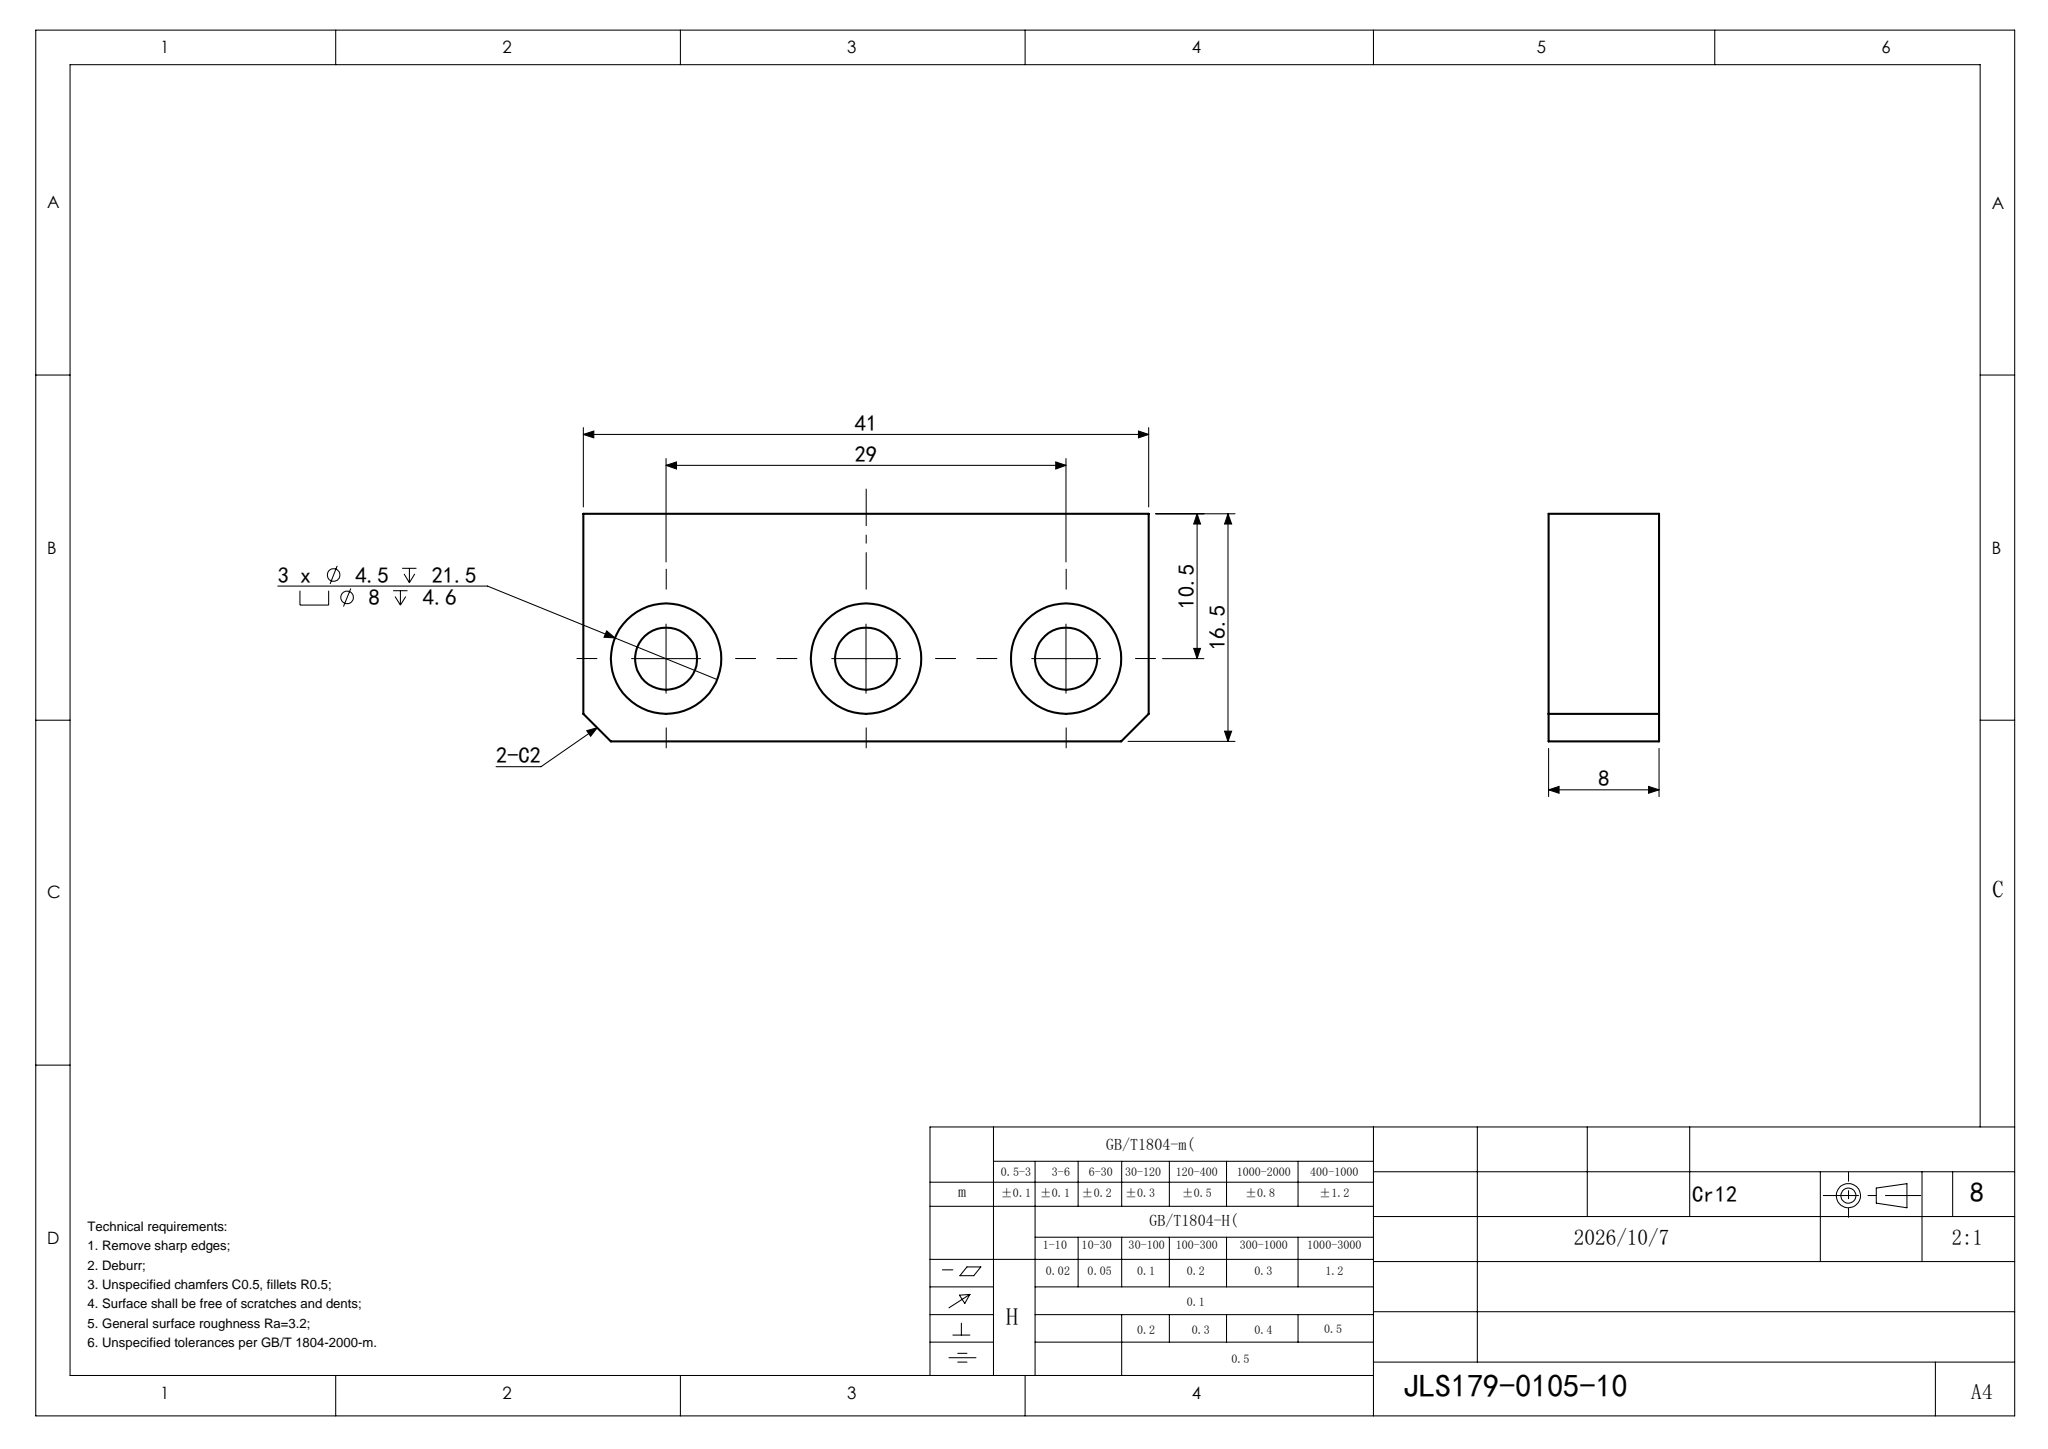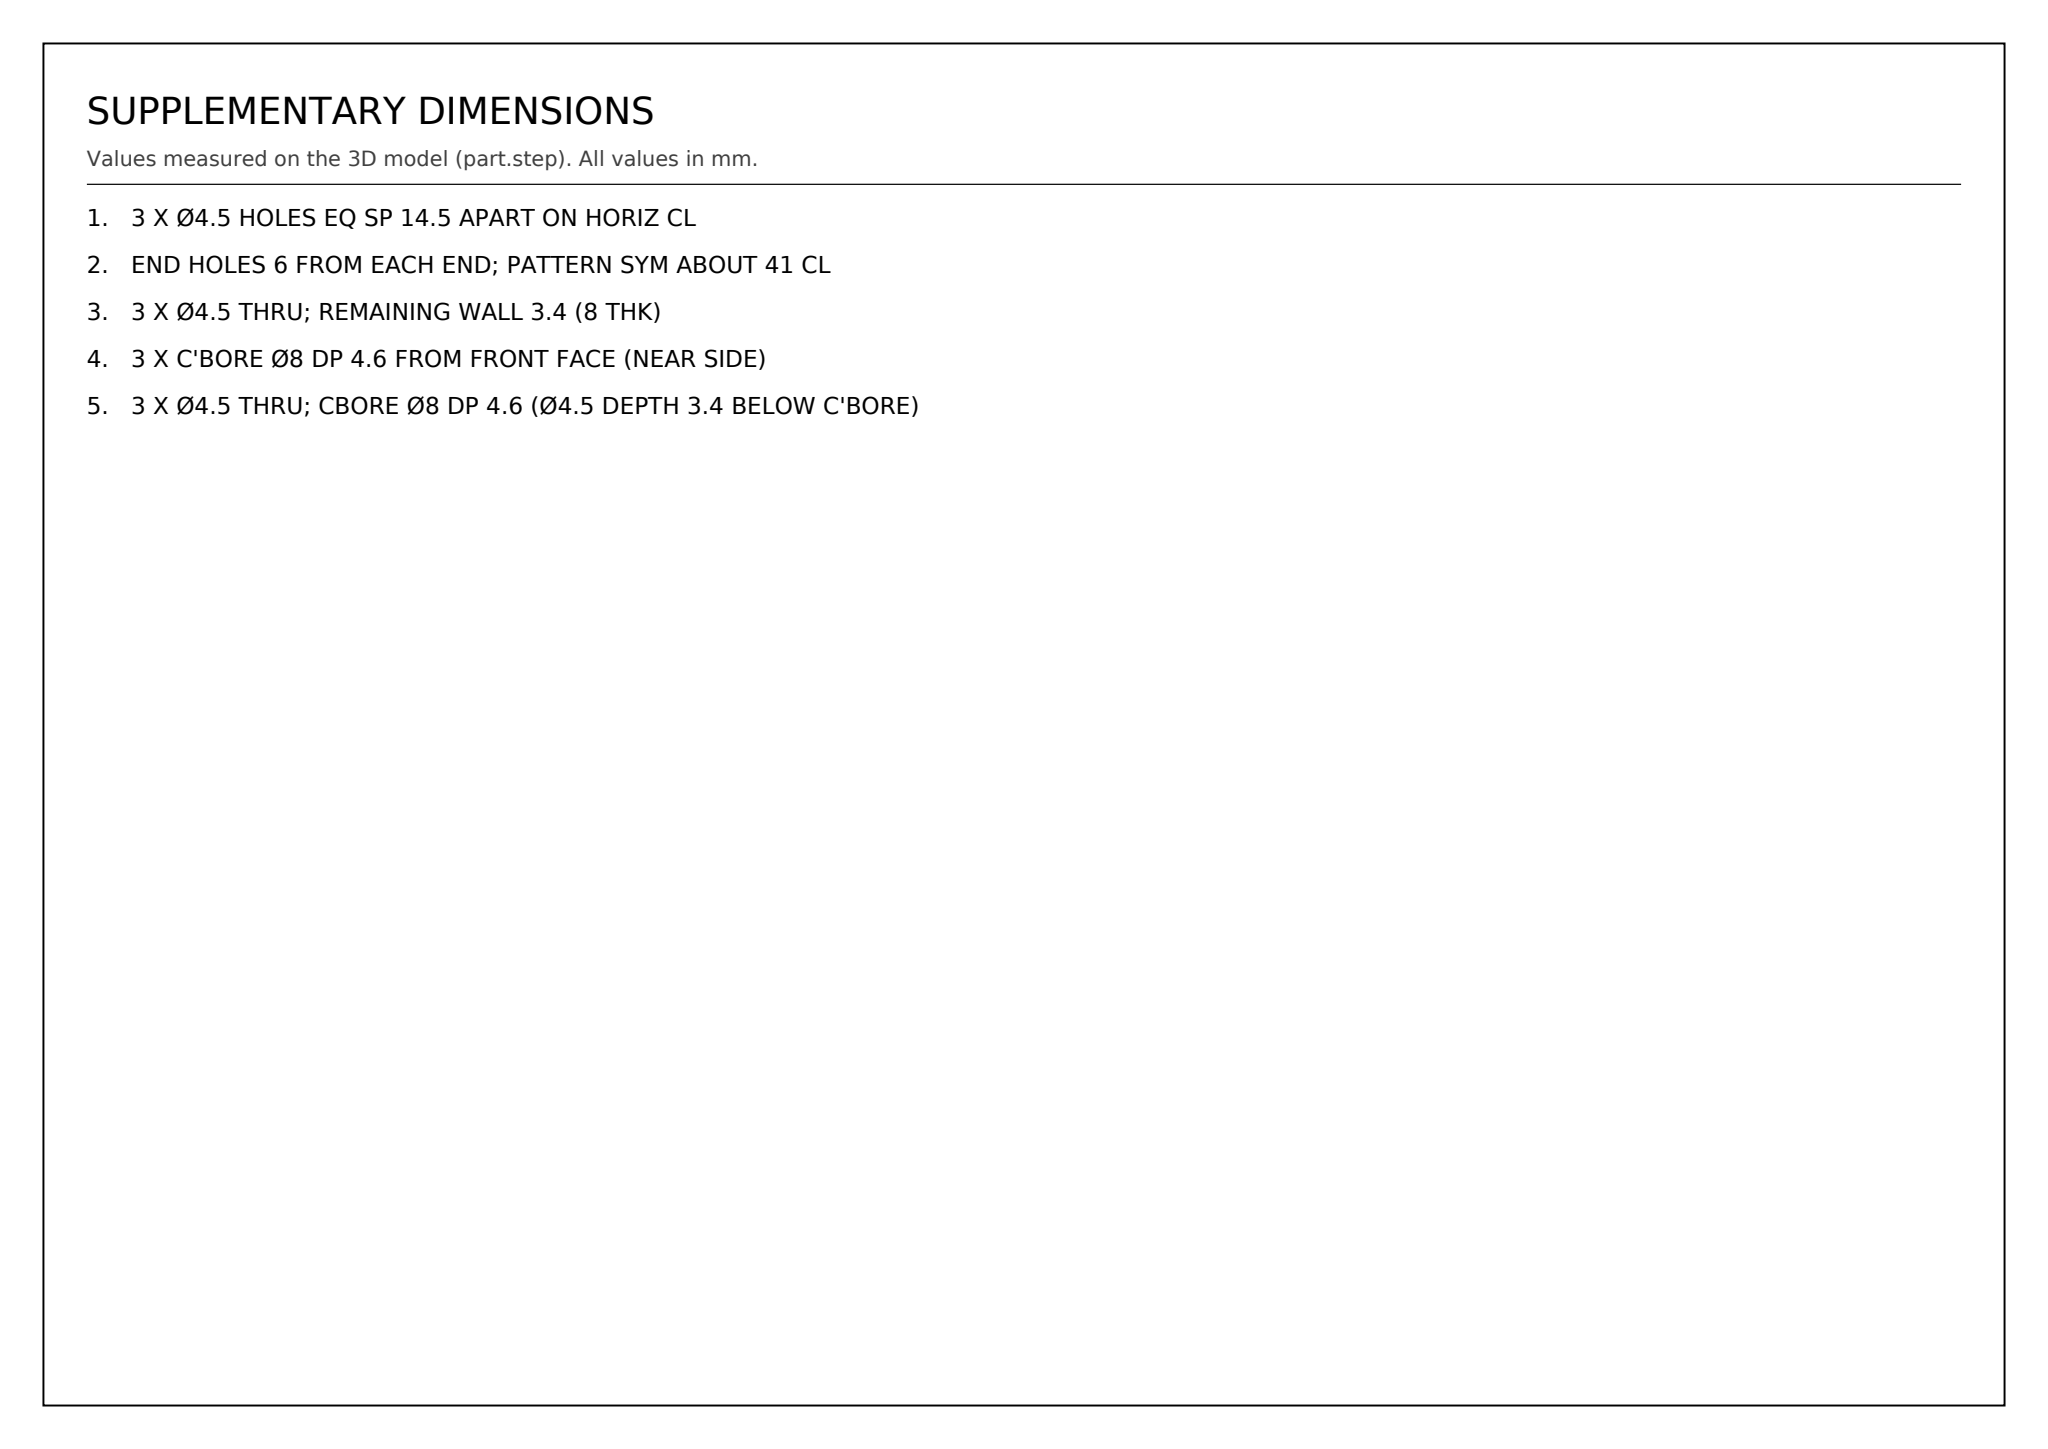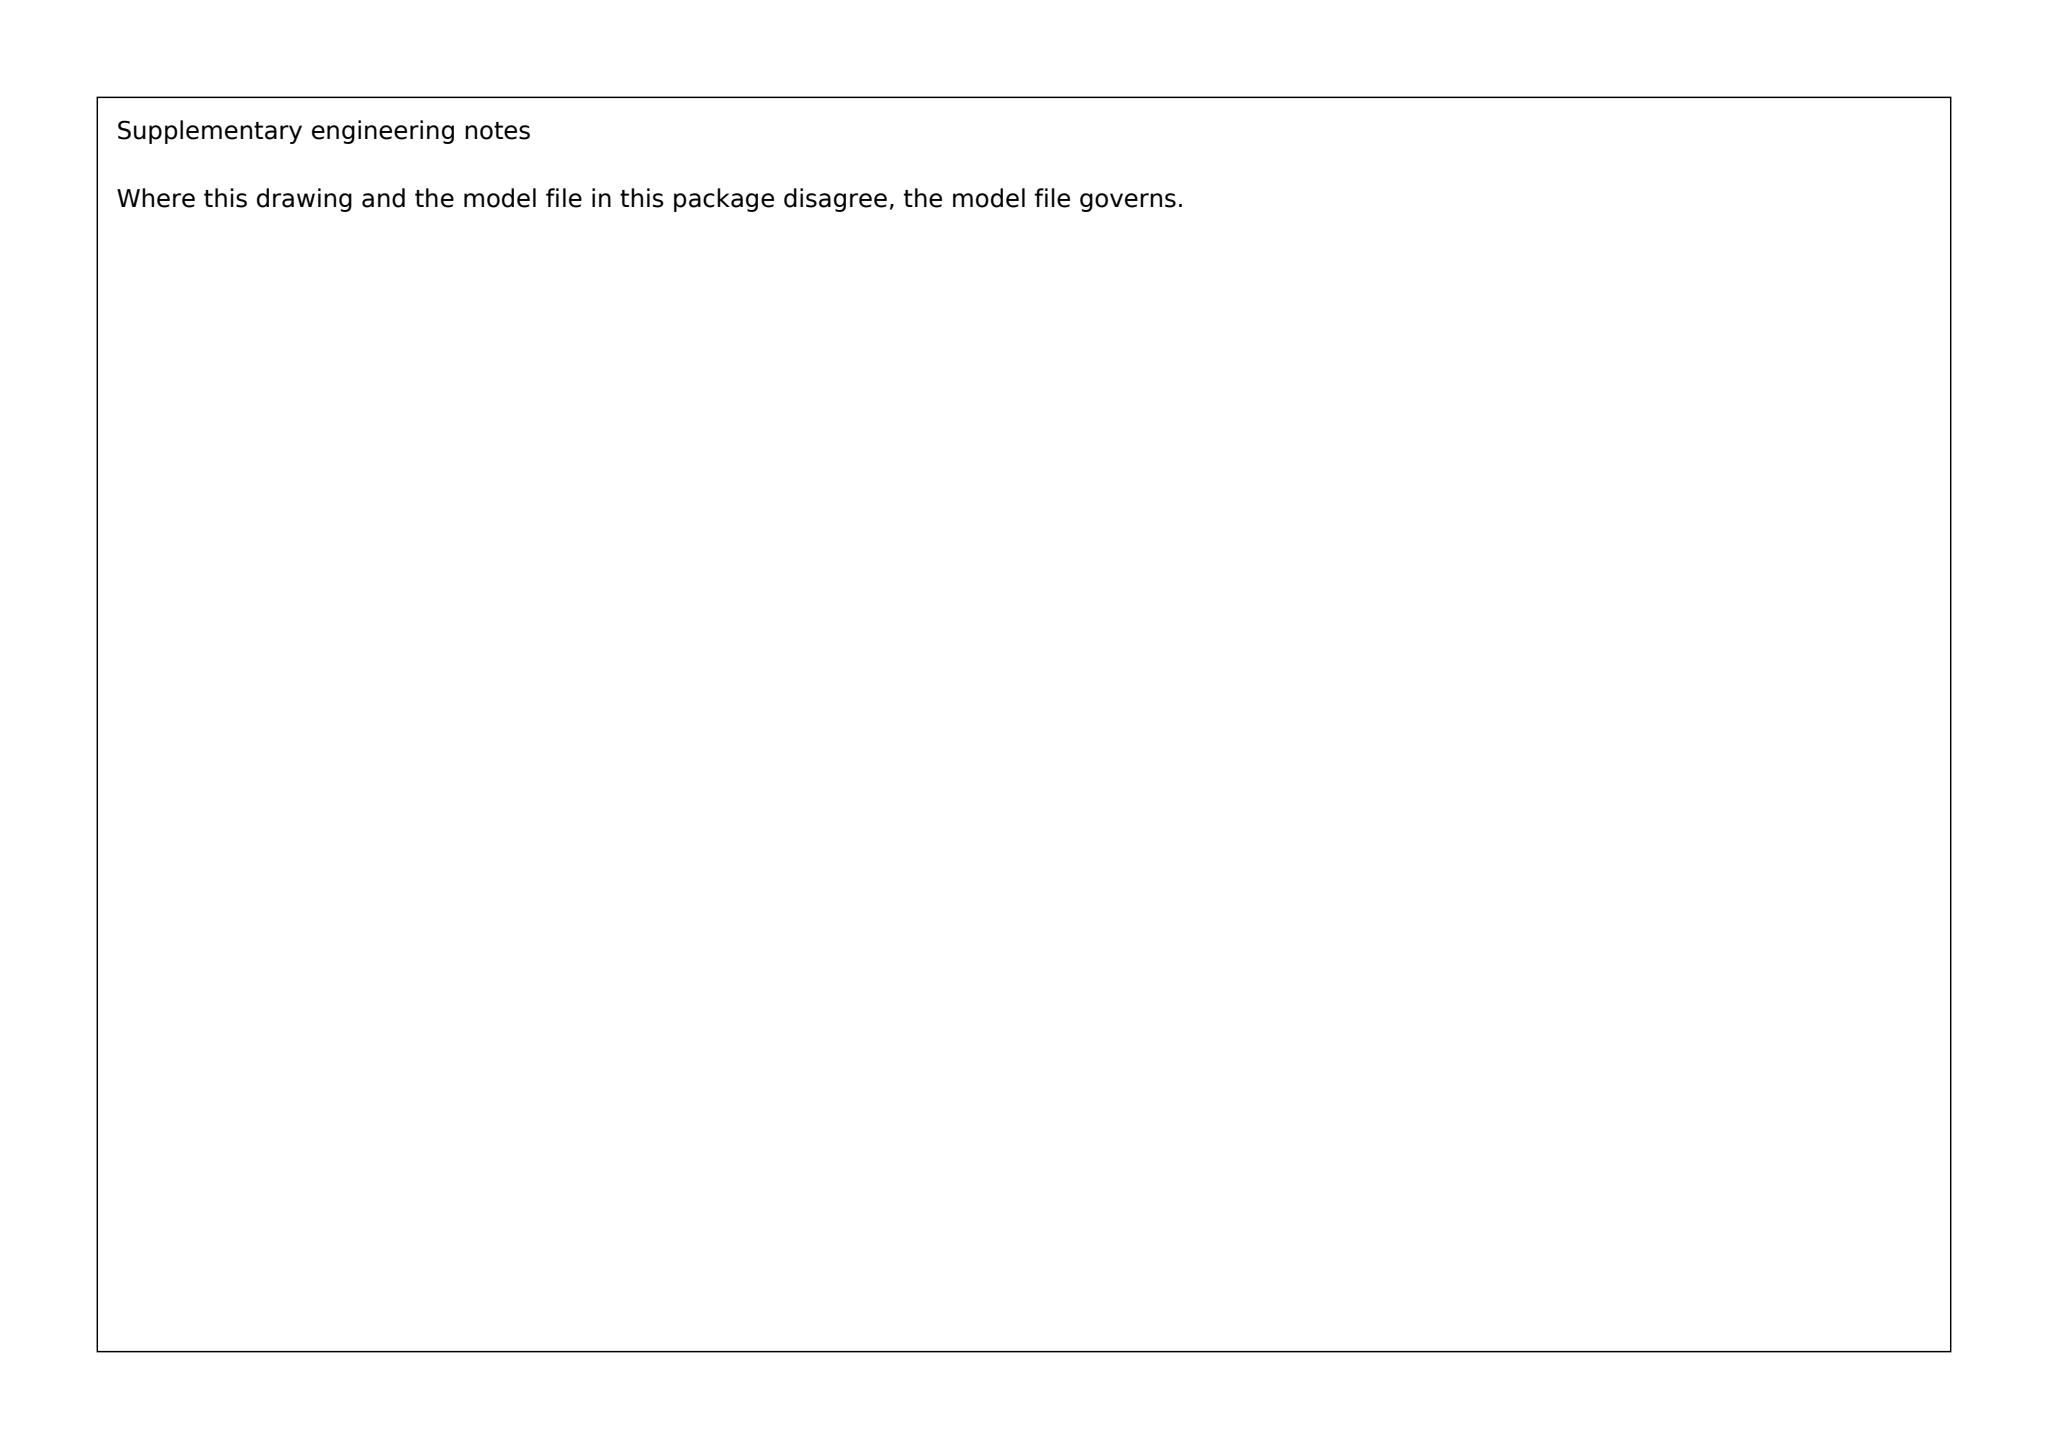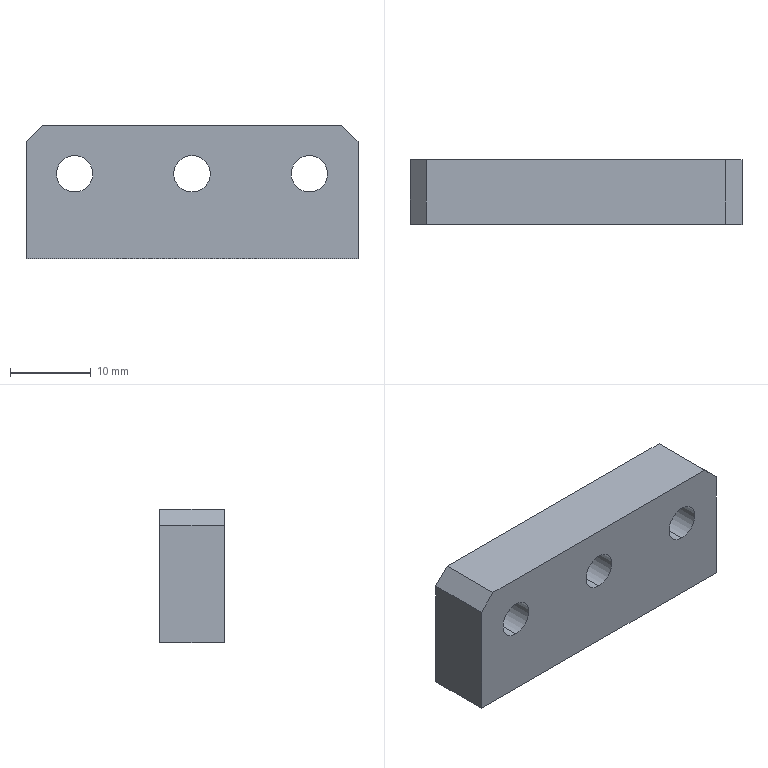Part | SolidWorks | mm | 1 solid | 23 faces | box 41 x 8 x 16.5 mm | volume 4524 mm3 | cylinder 12 | plane 11 | commonest cylinder face diameters 8 x6 4.5 x6
Drawing notes:
3 X Ø4.5 HOLES EQ SP 14.5 APART ON HORIZ CL | from the solid: Hole axes at x=6.0, 20.5, 35.0 -> 14.5 pitch, all z=10.5
END HOLES 6 FROM EACH END; PATTERN SYM ABOUT 41 CL | from the solid: x=6.0 and x=35.0 in 41.0 bbox; 41-35=6
3 X Ø4.5 THRU; REMAINING WALL 3.4 (8 THK) | from the solid: Ø4.5 length 3.4 from y=0 to y=3.4; bbox y=8.0
3 X C'BORE Ø8 DP 4.6 FROM FRONT FACE (NEAR SIDE) | from the solid: Ø8 length 4.6 from y=8.0 face down to y=3.4 plane
3 X Ø4.5 THRU; CBORE Ø8 DP 4.6 (Ø4.5 DEPTH 3.4 BELOW C'BORE) | from the solid: Ø4.5 cyl len 3.4 from y=3.4 to y=0; Ø8 cyl len 4.6 from y=8 to y=3.4; plate thk 8.0
build123d program:
from build123d import *

# Parameters (mm, degrees)
SKETCH1_W                                       = 41
SKETCH1_H                                       = 16.5
BOSS_EXTRUDE1_DEPTH                             = 8
M4_HEX_SOCKET_HEAD_CAP_SCREW_CBORE2_D           = 4.5
M4_HEX_SOCKET_HEAD_CAP_SCREW_CBORE2_DEPTH       = 21.5
M4_HEX_SOCKET_HEAD_CAP_SCREW_CBORE2_CBORE_D     = 8
M4_HEX_SOCKET_HEAD_CAP_SCREW_CBORE2_CBORE_DEPTH = 4.6
M4_HEX_SOCKET_HEAD_CAP_SCREW_CBORE2_TIP         = 1.352
CHAMFER1_SIZE                                   = 2


with BuildPart() as part:
    # Sketch1 → Boss-Extrude1 (new body)
    with BuildSketch(Plane(origin=(0, 0, 0), x_dir=(1, 0, 0), z_dir=(0, 1, 0))):
        Rectangle(SKETCH1_W, SKETCH1_H)
    extrude(amount=BOSS_EXTRUDE1_DEPTH)

    # M4 Hex Socket Head Cap Screw CBORE2
    with Locations(Plane(origin=(0, 8, 0), x_dir=(1, 0, 0), z_dir=(0, 1, 0))):
        with Locations((-14.5, -2.25), (14.5, -2.25), (0, -2.25)):
            CounterBoreHole(M4_HEX_SOCKET_HEAD_CAP_SCREW_CBORE2_D / 2, M4_HEX_SOCKET_HEAD_CAP_SCREW_CBORE2_CBORE_D / 2, M4_HEX_SOCKET_HEAD_CAP_SCREW_CBORE2_CBORE_DEPTH, depth=M4_HEX_SOCKET_HEAD_CAP_SCREW_CBORE2_DEPTH)
            with Locations((0, 0, -(M4_HEX_SOCKET_HEAD_CAP_SCREW_CBORE2_DEPTH + M4_HEX_SOCKET_HEAD_CAP_SCREW_CBORE2_TIP / 2))):  # 118° drill point
                Cone(0, M4_HEX_SOCKET_HEAD_CAP_SCREW_CBORE2_D / 2, M4_HEX_SOCKET_HEAD_CAP_SCREW_CBORE2_TIP, mode=Mode.SUBTRACT)

    # Chamfer1
    chamfer1_edges = [part.edges().sort_by_distance(p)[0] for p in [
        (20.5, 4, 8.25),
        (-20.5, 4, 8.25),
    ]]
    chamfer(chamfer1_edges, length=CHAMFER1_SIZE)


solid = part.part
STEP:
#1=CARTESIAN_POINT('',(-14.5,3.4,-1.75));
#2=VERTEX_POINT('',#1);
#3=CARTESIAN_POINT('',(-14.5,3.4,6.25));
#4=VERTEX_POINT('',#3);
#5=CARTESIAN_POINT('',(-14.5,3.4,2.25));
#6=DIRECTION('',(0.,1.,0.));
#7=DIRECTION('',(0.,0.,1.));
#8=AXIS2_PLACEMENT_3D('',#5,#6,#7);
#9=CIRCLE('',#8,4.);
#10=EDGE_CURVE('',#2,#4,#9,.T.);
#11=ORIENTED_EDGE('',*,*,#10,.F.);
#12=CARTESIAN_POINT('',(-14.5,8.,-1.75));
#13=VERTEX_POINT('',#12);
#14=CARTESIAN_POINT('',(-14.5,8.,-1.75));
#15=DIRECTION('',(0.,1.,0.));
#16=VECTOR('',#15,1000.);
#17=LINE('',#14,#16);
#18=EDGE_CURVE('',#2,#13,#17,.T.);
#19=ORIENTED_EDGE('',*,*,#18,.T.);
#20=CARTESIAN_POINT('',(-14.5,8.,6.25));
#21=VERTEX_POINT('',#20);
#22=CARTESIAN_POINT('',(-14.5,8.,2.25));
#23=DIRECTION('',(0.,1.,0.));
#24=DIRECTION('',(0.,0.,1.));
#25=AXIS2_PLACEMENT_3D('',#22,#23,#24);
#26=CIRCLE('',#25,4.);
#27=EDGE_CURVE('',#13,#21,#26,.T.);
#28=ORIENTED_EDGE('',*,*,#27,.T.);
#29=CARTESIAN_POINT('',(-14.5,8.,6.25));
#30=DIRECTION('',(0.,1.,0.));
#31=VECTOR('',#30,1000.);
#32=LINE('',#29,#31);
#33=EDGE_CURVE('',#4,#21,#32,.T.);
#34=ORIENTED_EDGE('',*,*,#33,.F.);
#35=EDGE_LOOP('',(#11,#19,#28,#34));
#36=FACE_OUTER_BOUND('',#35,.T.);
#37=CARTESIAN_POINT('',(-14.5,8.,2.25));
#38=DIRECTION('',(0.,1.,0.));
#39=DIRECTION('',(0.,0.,1.));
#40=AXIS2_PLACEMENT_3D('',#37,#38,#39);
#41=CYLINDRICAL_SURFACE('',#40,4.);
#42=ADVANCED_FACE('',(#36),#41,.F.);
#43=CARTESIAN_POINT('',(-14.5,0.,0.));
#44=VERTEX_POINT('',#43);
#45=CARTESIAN_POINT('',(-14.5,0.,4.5));
#46=VERTEX_POINT('',#45);
#47=CARTESIAN_POINT('',(-14.5,0.,2.25));
#48=DIRECTION('',(0.,1.,0.));
#49=DIRECTION('',(0.,0.,1.));
#50=AXIS2_PLACEMENT_3D('',#47,#48,#49);
#51=CIRCLE('',#50,2.25);
#52=EDGE_CURVE('',#44,#46,#51,.T.);
#53=ORIENTED_EDGE('',*,*,#52,.F.);
#54=CARTESIAN_POINT('',(-14.5,3.4,0.));
#55=VERTEX_POINT('',#54);
#56=CARTESIAN_POINT('',(-14.5,8.,0.));
#57=DIRECTION('',(0.,1.,0.));
#58=VECTOR('',#57,1000.);
#59=LINE('',#56,#58);
#60=EDGE_CURVE('',#44,#55,#59,.T.);
#61=ORIENTED_EDGE('',*,*,#60,.T.);
#62=CARTESIAN_POINT('',(-14.5,3.4,4.5));
#63=VERTEX_POINT('',#62);
#64=CARTESIAN_POINT('',(-14.5,3.4,2.25));
#65=DIRECTION('',(0.,1.,0.));
#66=DIRECTION('',(0.,0.,1.));
#67=AXIS2_PLACEMENT_3D('',#64,#65,#66);
#68=CIRCLE('',#67,2.25);
#69=EDGE_CURVE('',#55,#63,#68,.T.);
#70=ORIENTED_EDGE('',*,*,#69,.T.);
#71=CARTESIAN_POINT('',(-14.5,8.,4.5));
#72=DIRECTION('',(0.,1.,0.));
#73=VECTOR('',#72,1000.);
#74=LINE('',#71,#73);
#75=EDGE_CURVE('',#46,#63,#74,.T.);
#76=ORIENTED_EDGE('',*,*,#75,.F.);
#77=EDGE_LOOP('',(#53,#61,#70,#76));
#78=FACE_OUTER_BOUND('',#77,.T.);
#79=CARTESIAN_POINT('',(-14.5,8.,2.25));
#80=DIRECTION('',(0.,1.,0.));
#81=DIRECTION('',(0.,0.,1.));
#82=AXIS2_PLACEMENT_3D('',#79,#80,#81);
#83=CYLINDRICAL_SURFACE('',#82,2.25);
#84=ADVANCED_FACE('',(#78),#83,.F.);
#85=CARTESIAN_POINT('',(14.5,3.4,-1.75));
#86=VERTEX_POINT('',#85);
#87=CARTESIAN_POINT('',(14.5,3.4,6.25));
#88=VERTEX_POINT('',#87);
#89=CARTESIAN_POINT('',(14.5,3.4,2.25));
#90=DIRECTION('',(0.,1.,0.));
#91=DIRECTION('',(0.,0.,1.));
#92=AXIS2_PLACEMENT_3D('',#89,#90,#91);
#93=CIRCLE('',#92,4.);
#94=EDGE_CURVE('',#86,#88,#93,.T.);
#95=ORIENTED_EDGE('',*,*,#94,.F.);
#96=CARTESIAN_POINT('',(14.5,8.,-1.75));
#97=VERTEX_POINT('',#96);
#98=CARTESIAN_POINT('',(14.5,8.,-1.75));
#99=DIRECTION('',(0.,1.,0.));
#100=VECTOR('',#99,1000.);
#101=LINE('',#98,#100);
#102=EDGE_CURVE('',#86,#97,#101,.T.);
#103=ORIENTED_EDGE('',*,*,#102,.T.);
#104=CARTESIAN_POINT('',(14.5,8.,6.25));
#105=VERTEX_POINT('',#104);
#106=CARTESIAN_POINT('',(14.5,8.,2.25));
#107=DIRECTION('',(0.,1.,0.));
#108=DIRECTION('',(0.,0.,1.));
#109=AXIS2_PLACEMENT_3D('',#106,#107,#108);
#110=CIRCLE('',#109,4.);
#111=EDGE_CURVE('',#97,#105,#110,.T.);
#112=ORIENTED_EDGE('',*,*,#111,.T.);
#113=CARTESIAN_POINT('',(14.5,8.,6.25));
#114=DIRECTION('',(0.,1.,0.));
#115=VECTOR('',#114,1000.);
#116=LINE('',#113,#115);
#117=EDGE_CURVE('',#88,#105,#116,.T.);
#118=ORIENTED_EDGE('',*,*,#117,.F.);
#119=EDGE_LOOP('',(#95,#103,#112,#118));
#120=FACE_OUTER_BOUND('',#119,.T.);
#121=CARTESIAN_POINT('',(14.5,8.,2.25));
#122=DIRECTION('',(0.,1.,0.));
#123=DIRECTION('',(0.,0.,1.));
#124=AXIS2_PLACEMENT_3D('',#121,#122,#123);
#125=CYLINDRICAL_SURFACE('',#124,4.);
#126=ADVANCED_FACE('',(#120),#125,.F.);
#127=CARTESIAN_POINT('',(14.5,0.,0.));
#128=VERTEX_POINT('',#127);
#129=CARTESIAN_POINT('',(14.5,0.,4.5));
#130=VERTEX_POINT('',#129);
#131=CARTESIAN_POINT('',(14.5,0.,2.25));
#132=DIRECTION('',(0.,1.,0.));
#133=DIRECTION('',(0.,0.,1.));
#134=AXIS2_PLACEMENT_3D('',#131,#132,#133);
#135=CIRCLE('',#134,2.25);
#136=EDGE_CURVE('',#128,#130,#135,.T.);
#137=ORIENTED_EDGE('',*,*,#136,.F.);
#138=CARTESIAN_POINT('',(14.5,3.4,0.));
#139=VERTEX_POINT('',#138);
#140=CARTESIAN_POINT('',(14.5,8.,0.));
#141=DIRECTION('',(0.,1.,0.));
#142=VECTOR('',#141,1000.);
#143=LINE('',#140,#142);
#144=EDGE_CURVE('',#128,#139,#143,.T.);
#145=ORIENTED_EDGE('',*,*,#144,.T.);
#146=CARTESIAN_POINT('',(14.5,3.4,4.5));
#147=VERTEX_POINT('',#146);
#148=CARTESIAN_POINT('',(14.5,3.4,2.25));
#149=DIRECTION('',(0.,1.,0.));
#150=DIRECTION('',(0.,0.,1.));
#151=AXIS2_PLACEMENT_3D('',#148,#149,#150);
#152=CIRCLE('',#151,2.25);
#153=EDGE_CURVE('',#139,#147,#152,.T.);
#154=ORIENTED_EDGE('',*,*,#153,.T.);
#155=CARTESIAN_POINT('',(14.5,8.,4.5));
#156=DIRECTION('',(0.,1.,0.));
#157=VECTOR('',#156,1000.);
#158=LINE('',#155,#157);
#159=EDGE_CURVE('',#130,#147,#158,.T.);
#160=ORIENTED_EDGE('',*,*,#159,.F.);
#161=EDGE_LOOP('',(#137,#145,#154,#160));
#162=FACE_OUTER_BOUND('',#161,.T.);
#163=CARTESIAN_POINT('',(14.5,8.,2.25));
#164=DIRECTION('',(0.,1.,0.));
#165=DIRECTION('',(0.,0.,1.));
#166=AXIS2_PLACEMENT_3D('',#163,#164,#165);
#167=CYLINDRICAL_SURFACE('',#166,2.25);
#168=ADVANCED_FACE('',(#162),#167,.F.);
#169=CARTESIAN_POINT('',(0.,3.4,-1.75));
#170=VERTEX_POINT('',#169);
#171=CARTESIAN_POINT('',(0.,3.4,6.25));
#172=VERTEX_POINT('',#171);
#173=CARTESIAN_POINT('',(0.,3.4,2.25));
#174=DIRECTION('',(0.,1.,0.));
#175=DIRECTION('',(0.,0.,1.));
#176=AXIS2_PLACEMENT_3D('',#173,#174,#175);
#177=CIRCLE('',#176,4.);
#178=EDGE_CURVE('',#170,#172,#177,.T.);
#179=ORIENTED_EDGE('',*,*,#178,.F.);
#180=CARTESIAN_POINT('',(0.,8.,-1.75));
#181=VERTEX_POINT('',#180);
#182=CARTESIAN_POINT('',(0.,8.,-1.75));
#183=DIRECTION('',(0.,1.,0.));
#184=VECTOR('',#183,1000.);
#185=LINE('',#182,#184);
#186=EDGE_CURVE('',#170,#181,#185,.T.);
#187=ORIENTED_EDGE('',*,*,#186,.T.);
#188=CARTESIAN_POINT('',(0.,8.,6.25));
#189=VERTEX_POINT('',#188);
#190=CARTESIAN_POINT('',(0.,8.,2.25));
#191=DIRECTION('',(0.,1.,0.));
#192=DIRECTION('',(0.,0.,1.));
#193=AXIS2_PLACEMENT_3D('',#190,#191,#192);
#194=CIRCLE('',#193,4.);
#195=EDGE_CURVE('',#181,#189,#194,.T.);
#196=ORIENTED_EDGE('',*,*,#195,.T.);
#197=CARTESIAN_POINT('',(0.,8.,6.25));
#198=DIRECTION('',(0.,1.,0.));
#199=VECTOR('',#198,1000.);
#200=LINE('',#197,#199);
#201=EDGE_CURVE('',#172,#189,#200,.T.);
#202=ORIENTED_EDGE('',*,*,#201,.F.);
#203=EDGE_LOOP('',(#179,#187,#196,#202));
#204=FACE_OUTER_BOUND('',#203,.T.);
#205=CARTESIAN_POINT('',(0.,8.,2.25));
#206=DIRECTION('',(0.,1.,0.));
#207=DIRECTION('',(0.,0.,1.));
#208=AXIS2_PLACEMENT_3D('',#205,#206,#207);
#209=CYLINDRICAL_SURFACE('',#208,4.);
#210=ADVANCED_FACE('',(#204),#209,.F.);
#211=CARTESIAN_POINT('',(0.,0.,0.));
#212=VERTEX_POINT('',#211);
#213=CARTESIAN_POINT('',(0.,0.,4.5));
#214=VERTEX_POINT('',#213);
#215=CARTESIAN_POINT('',(0.,0.,2.25));
#216=DIRECTION('',(0.,1.,0.));
#217=DIRECTION('',(0.,0.,1.));
#218=AXIS2_PLACEMENT_3D('',#215,#216,#217);
#219=CIRCLE('',#218,2.25);
#220=EDGE_CURVE('',#212,#214,#219,.T.);
#221=ORIENTED_EDGE('',*,*,#220,.F.);
#222=CARTESIAN_POINT('',(0.,3.4,0.));
#223=VERTEX_POINT('',#222);
#224=CARTESIAN_POINT('',(0.,8.,0.));
#225=DIRECTION('',(0.,1.,0.));
#226=VECTOR('',#225,1000.);
#227=LINE('',#224,#226);
#228=EDGE_CURVE('',#212,#223,#227,.T.);
#229=ORIENTED_EDGE('',*,*,#228,.T.);
#230=CARTESIAN_POINT('',(0.,3.4,4.5));
#231=VERTEX_POINT('',#230);
#232=CARTESIAN_POINT('',(0.,3.4,2.25));
#233=DIRECTION('',(0.,1.,0.));
#234=DIRECTION('',(0.,0.,1.));
#235=AXIS2_PLACEMENT_3D('',#232,#233,#234);
#236=CIRCLE('',#235,2.25);
#237=EDGE_CURVE('',#223,#231,#236,.T.);
#238=ORIENTED_EDGE('',*,*,#237,.T.);
#239=CARTESIAN_POINT('',(0.,8.,4.5));
#240=DIRECTION('',(0.,1.,0.));
#241=VECTOR('',#240,1000.);
#242=LINE('',#239,#241);
#243=EDGE_CURVE('',#214,#231,#242,.T.);
#244=ORIENTED_EDGE('',*,*,#243,.F.);
#245=EDGE_LOOP('',(#221,#229,#238,#244));
#246=FACE_OUTER_BOUND('',#245,.T.);
#247=CARTESIAN_POINT('',(0.,8.,2.25));
#248=DIRECTION('',(0.,1.,0.));
#249=DIRECTION('',(0.,0.,1.));
#250=AXIS2_PLACEMENT_3D('',#247,#248,#249);
#251=CYLINDRICAL_SURFACE('',#250,2.25);
#252=ADVANCED_FACE('',(#246),#251,.F.);
#253=CARTESIAN_POINT('',(-20.5,0.,-8.25));
#254=VERTEX_POINT('',#253);
#255=CARTESIAN_POINT('',(-20.5,0.,6.25));
#256=VERTEX_POINT('',#255);
#257=CARTESIAN_POINT('',(-20.5,0.,8.25));
#258=DIRECTION('',(0.,0.,1.));
#259=VECTOR('',#258,1000.);
#260=LINE('',#257,#259);
#261=EDGE_CURVE('',#254,#256,#260,.T.);
#262=ORIENTED_EDGE('',*,*,#261,.T.);
#263=CARTESIAN_POINT('',(-20.5,8.,6.25));
#264=VERTEX_POINT('',#263);
#265=CARTESIAN_POINT('',(-20.5,8.,6.25));
#266=DIRECTION('',(0.,1.,0.));
#267=VECTOR('',#266,1000.);
#268=LINE('',#265,#267);
#269=EDGE_CURVE('',#256,#264,#268,.T.);
#270=ORIENTED_EDGE('',*,*,#269,.T.);
#271=CARTESIAN_POINT('',(-20.5,8.,-8.25));
#272=VERTEX_POINT('',#271);
#273=CARTESIAN_POINT('',(-20.5,8.,8.25));
#274=DIRECTION('',(0.,0.,1.));
#275=VECTOR('',#274,1000.);
#276=LINE('',#273,#275);
#277=EDGE_CURVE('',#272,#264,#276,.T.);
#278=ORIENTED_EDGE('',*,*,#277,.F.);
#279=CARTESIAN_POINT('',(-20.5,8.,-8.25));
#280=DIRECTION('',(0.,-1.,0.));
#281=VECTOR('',#280,1000.);
#282=LINE('',#279,#281);
#283=EDGE_CURVE('',#272,#254,#282,.T.);
#284=ORIENTED_EDGE('',*,*,#283,.T.);
#285=EDGE_LOOP('',(#262,#270,#278,#284));
#286=FACE_OUTER_BOUND('',#285,.T.);
#287=CARTESIAN_POINT('',(-20.5,8.,8.25));
#288=DIRECTION('',(1.,0.,0.));
#289=DIRECTION('',(0.,0.,-1.));
#290=AXIS2_PLACEMENT_3D('',#287,#288,#289);
#291=PLANE('',#290);
#292=ADVANCED_FACE('',(#286),#291,.F.);
#293=CARTESIAN_POINT('',(-18.5,0.,8.25));
#294=VERTEX_POINT('',#293);
#295=CARTESIAN_POINT('',(18.5,0.,8.25));
#296=VERTEX_POINT('',#295);
#297=CARTESIAN_POINT('',(20.5,0.,8.25));
#298=DIRECTION('',(1.,0.,-0.));
#299=VECTOR('',#298,1000.);
#300=LINE('',#297,#299);
#301=EDGE_CURVE('',#294,#296,#300,.T.);
#302=ORIENTED_EDGE('',*,*,#301,.T.);
#303=CARTESIAN_POINT('',(18.5,8.,8.25));
#304=VERTEX_POINT('',#303);
#305=CARTESIAN_POINT('',(18.5,8.,8.25));
#306=DIRECTION('',(0.,1.,0.));
#307=VECTOR('',#306,1000.);
#308=LINE('',#305,#307);
#309=EDGE_CURVE('',#296,#304,#308,.T.);
#310=ORIENTED_EDGE('',*,*,#309,.T.);
#311=CARTESIAN_POINT('',(-18.5,8.,8.25));
#312=VERTEX_POINT('',#311);
#313=CARTESIAN_POINT('',(20.5,8.,8.25));
#314=DIRECTION('',(1.,0.,-0.));
#315=VECTOR('',#314,1000.);
#316=LINE('',#313,#315);
#317=EDGE_CURVE('',#312,#304,#316,.T.);
#318=ORIENTED_EDGE('',*,*,#317,.F.);
#319=CARTESIAN_POINT('',(-18.5,8.,8.25));
#320=DIRECTION('',(0.,-1.,0.));
#321=VECTOR('',#320,1000.);
#322=LINE('',#319,#321);
#323=EDGE_CURVE('',#312,#294,#322,.T.);
#324=ORIENTED_EDGE('',*,*,#323,.T.);
#325=EDGE_LOOP('',(#302,#310,#318,#324));
#326=FACE_OUTER_BOUND('',#325,.T.);
#327=CARTESIAN_POINT('',(20.5,8.,8.25));
#328=DIRECTION('',(-0.,0.,-1.));
#329=DIRECTION('',(-1.,0.,0.));
#330=AXIS2_PLACEMENT_3D('',#327,#328,#329);
#331=PLANE('',#330);
#332=ADVANCED_FACE('',(#326),#331,.F.);
#333=CARTESIAN_POINT('',(20.5,8.,6.25));
#334=VERTEX_POINT('',#333);
#335=CARTESIAN_POINT('',(20.5,8.,-8.25));
#336=VERTEX_POINT('',#335);
#337=CARTESIAN_POINT('',(20.5,8.,8.25));
#338=DIRECTION('',(0.,0.,-1.));
#339=VECTOR('',#338,1000.);
#340=LINE('',#337,#339);
#341=EDGE_CURVE('',#334,#336,#340,.T.);
#342=ORIENTED_EDGE('',*,*,#341,.F.);
#343=CARTESIAN_POINT('',(20.5,0.,6.25));
#344=VERTEX_POINT('',#343);
#345=CARTESIAN_POINT('',(20.5,8.,6.25));
#346=DIRECTION('',(0.,-1.,0.));
#347=VECTOR('',#346,1000.);
#348=LINE('',#345,#347);
#349=EDGE_CURVE('',#334,#344,#348,.T.);
#350=ORIENTED_EDGE('',*,*,#349,.T.);
#351=CARTESIAN_POINT('',(20.5,0.,-8.25));
#352=VERTEX_POINT('',#351);
#353=CARTESIAN_POINT('',(20.5,0.,8.25));
#354=DIRECTION('',(0.,0.,-1.));
#355=VECTOR('',#354,1000.);
#356=LINE('',#353,#355);
#357=EDGE_CURVE('',#344,#352,#356,.T.);
#358=ORIENTED_EDGE('',*,*,#357,.T.);
#359=CARTESIAN_POINT('',(20.5,8.,-8.25));
#360=DIRECTION('',(0.,-1.,0.));
#361=VECTOR('',#360,1000.);
#362=LINE('',#359,#361);
#363=EDGE_CURVE('',#336,#352,#362,.T.);
#364=ORIENTED_EDGE('',*,*,#363,.F.);
#365=EDGE_LOOP('',(#342,#350,#358,#364));
#366=FACE_OUTER_BOUND('',#365,.T.);
#367=CARTESIAN_POINT('',(20.5,8.,8.25));
#368=DIRECTION('',(-1.,0.,0.));
#369=DIRECTION('',(0.,0.,1.));
#370=AXIS2_PLACEMENT_3D('',#367,#368,#369);
#371=PLANE('',#370);
#372=ADVANCED_FACE('',(#366),#371,.F.);
#373=CARTESIAN_POINT('',(20.5,0.,-8.25));
#374=DIRECTION('',(-1.,0.,0.));
#375=VECTOR('',#374,1000.);
#376=LINE('',#373,#375);
#377=EDGE_CURVE('',#352,#254,#376,.T.);
#378=ORIENTED_EDGE('',*,*,#377,.T.);
#379=ORIENTED_EDGE('',*,*,#283,.F.);
#380=CARTESIAN_POINT('',(20.5,8.,-8.25));
#381=DIRECTION('',(-1.,0.,0.));
#382=VECTOR('',#381,1000.);
#383=LINE('',#380,#382);
#384=EDGE_CURVE('',#336,#272,#383,.T.);
#385=ORIENTED_EDGE('',*,*,#384,.F.);
#386=ORIENTED_EDGE('',*,*,#363,.T.);
#387=EDGE_LOOP('',(#378,#379,#385,#386));
#388=FACE_OUTER_BOUND('',#387,.T.);
#389=CARTESIAN_POINT('',(20.5,8.,-8.25));
#390=DIRECTION('',(0.,0.,1.));
#391=DIRECTION('',(1.,0.,-0.));
#392=AXIS2_PLACEMENT_3D('',#389,#390,#391);
#393=PLANE('',#392);
#394=ADVANCED_FACE('',(#388),#393,.F.);
#395=CARTESIAN_POINT('',(-14.5,8.,2.25));
#396=DIRECTION('',(0.,1.,0.));
#397=DIRECTION('',(0.,0.,1.));
#398=AXIS2_PLACEMENT_3D('',#395,#396,#397);
#399=CIRCLE('',#398,4.);
#400=EDGE_CURVE('',#21,#13,#399,.T.);
#401=ORIENTED_EDGE('',*,*,#400,.F.);
#402=ORIENTED_EDGE('',*,*,#27,.F.);
#403=EDGE_LOOP('',(#401,#402));
#404=FACE_BOUND('',#403,.T.);
#405=CARTESIAN_POINT('',(14.5,8.,2.25));
#406=DIRECTION('',(0.,1.,0.));
#407=DIRECTION('',(0.,0.,1.));
#408=AXIS2_PLACEMENT_3D('',#405,#406,#407);
#409=CIRCLE('',#408,4.);
#410=EDGE_CURVE('',#105,#97,#409,.T.);
#411=ORIENTED_EDGE('',*,*,#410,.F.);
#412=ORIENTED_EDGE('',*,*,#111,.F.);
#413=EDGE_LOOP('',(#411,#412));
#414=FACE_BOUND('',#413,.T.);
#415=CARTESIAN_POINT('',(0.,8.,2.25));
#416=DIRECTION('',(0.,1.,0.));
#417=DIRECTION('',(0.,0.,1.));
#418=AXIS2_PLACEMENT_3D('',#415,#416,#417);
#419=CIRCLE('',#418,4.);
#420=EDGE_CURVE('',#189,#181,#419,.T.);
#421=ORIENTED_EDGE('',*,*,#420,.F.);
#422=ORIENTED_EDGE('',*,*,#195,.F.);
#423=EDGE_LOOP('',(#421,#422));
#424=FACE_BOUND('',#423,.T.);
#425=ORIENTED_EDGE('',*,*,#317,.T.);
#426=CARTESIAN_POINT('',(13.375,8.,13.375));
#427=DIRECTION('',(0.7071,0.,-0.7071));
#428=VECTOR('',#427,1000.);
#429=LINE('',#426,#428);
#430=EDGE_CURVE('',#304,#334,#429,.T.);
#431=ORIENTED_EDGE('',*,*,#430,.T.);
#432=ORIENTED_EDGE('',*,*,#341,.T.);
#433=ORIENTED_EDGE('',*,*,#384,.T.);
#434=ORIENTED_EDGE('',*,*,#277,.T.);
#435=CARTESIAN_POINT('',(-13.375,8.,13.375));
#436=DIRECTION('',(0.7071,0.,0.7071));
#437=VECTOR('',#436,1000.);
#438=LINE('',#435,#437);
#439=EDGE_CURVE('',#264,#312,#438,.T.);
#440=ORIENTED_EDGE('',*,*,#439,.T.);
#441=EDGE_LOOP('',(#425,#431,#432,#433,#434,#440));
#442=FACE_OUTER_BOUND('',#441,.T.);
#443=CARTESIAN_POINT('',(0.,8.,0.));
#444=DIRECTION('',(0.,1.,0.));
#445=DIRECTION('',(0.,0.,1.));
#446=AXIS2_PLACEMENT_3D('',#443,#444,#445);
#447=PLANE('',#446);
#448=ADVANCED_FACE('',(#404,#414,#424,#442),#447,.T.);
#449=CARTESIAN_POINT('',(-14.5,0.,2.25));
#450=DIRECTION('',(0.,1.,0.));
#451=DIRECTION('',(0.,0.,1.));
#452=AXIS2_PLACEMENT_3D('',#449,#450,#451);
#453=CIRCLE('',#452,2.25);
#454=EDGE_CURVE('',#46,#44,#453,.T.);
#455=ORIENTED_EDGE('',*,*,#454,.T.);
#456=ORIENTED_EDGE('',*,*,#52,.T.);
#457=EDGE_LOOP('',(#455,#456));
#458=FACE_BOUND('',#457,.T.);
#459=CARTESIAN_POINT('',(14.5,0.,2.25));
#460=DIRECTION('',(0.,1.,0.));
#461=DIRECTION('',(0.,0.,1.));
#462=AXIS2_PLACEMENT_3D('',#459,#460,#461);
#463=CIRCLE('',#462,2.25);
#464=EDGE_CURVE('',#130,#128,#463,.T.);
#465=ORIENTED_EDGE('',*,*,#464,.T.);
#466=ORIENTED_EDGE('',*,*,#136,.T.);
#467=EDGE_LOOP('',(#465,#466));
#468=FACE_BOUND('',#467,.T.);
#469=CARTESIAN_POINT('',(0.,0.,2.25));
#470=DIRECTION('',(0.,1.,0.));
#471=DIRECTION('',(0.,0.,1.));
#472=AXIS2_PLACEMENT_3D('',#469,#470,#471);
#473=CIRCLE('',#472,2.25);
#474=EDGE_CURVE('',#214,#212,#473,.T.);
#475=ORIENTED_EDGE('',*,*,#474,.T.);
#476=ORIENTED_EDGE('',*,*,#220,.T.);
#477=EDGE_LOOP('',(#475,#476));
#478=FACE_BOUND('',#477,.T.);
#479=ORIENTED_EDGE('',*,*,#357,.F.);
#480=CARTESIAN_POINT('',(20.5,0.,6.25));
#481=DIRECTION('',(-0.7071,0.,0.7071));
#482=VECTOR('',#481,1000.);
#483=LINE('',#480,#482);
#484=EDGE_CURVE('',#344,#296,#483,.T.);
#485=ORIENTED_EDGE('',*,*,#484,.T.);
#486=ORIENTED_EDGE('',*,*,#301,.F.);
#487=CARTESIAN_POINT('',(-18.5,0.,8.25));
#488=DIRECTION('',(-0.7071,0.,-0.7071));
#489=VECTOR('',#488,1000.);
#490=LINE('',#487,#489);
#491=EDGE_CURVE('',#294,#256,#490,.T.);
#492=ORIENTED_EDGE('',*,*,#491,.T.);
#493=ORIENTED_EDGE('',*,*,#261,.F.);
#494=ORIENTED_EDGE('',*,*,#377,.F.);
#495=EDGE_LOOP('',(#479,#485,#486,#492,#493,#494));
#496=FACE_OUTER_BOUND('',#495,.T.);
#497=CARTESIAN_POINT('',(0.,0.,0.));
#498=DIRECTION('',(0.,1.,0.));
#499=DIRECTION('',(0.,0.,1.));
#500=AXIS2_PLACEMENT_3D('',#497,#498,#499);
#501=PLANE('',#500);
#502=ADVANCED_FACE('',(#458,#468,#478,#496),#501,.F.);
#503=ORIENTED_EDGE('',*,*,#228,.F.);
#504=ORIENTED_EDGE('',*,*,#474,.F.);
#505=ORIENTED_EDGE('',*,*,#243,.T.);
#506=CARTESIAN_POINT('',(0.,3.4,2.25));
#507=DIRECTION('',(0.,1.,0.));
#508=DIRECTION('',(0.,0.,1.));
#509=AXIS2_PLACEMENT_3D('',#506,#507,#508);
#510=CIRCLE('',#509,2.25);
#511=EDGE_CURVE('',#231,#223,#510,.T.);
#512=ORIENTED_EDGE('',*,*,#511,.T.);
#513=EDGE_LOOP('',(#503,#504,#505,#512));
#514=FACE_OUTER_BOUND('',#513,.T.);
#515=CARTESIAN_POINT('',(0.,8.,2.25));
#516=DIRECTION('',(0.,1.,0.));
#517=DIRECTION('',(0.,0.,1.));
#518=AXIS2_PLACEMENT_3D('',#515,#516,#517);
#519=CYLINDRICAL_SURFACE('',#518,2.25);
#520=ADVANCED_FACE('',(#514),#519,.F.);
#521=ORIENTED_EDGE('',*,*,#511,.F.);
#522=ORIENTED_EDGE('',*,*,#237,.F.);
#523=EDGE_LOOP('',(#521,#522));
#524=FACE_BOUND('',#523,.T.);
#525=CARTESIAN_POINT('',(0.,3.4,2.25));
#526=DIRECTION('',(0.,1.,0.));
#527=DIRECTION('',(0.,0.,1.));
#528=AXIS2_PLACEMENT_3D('',#525,#526,#527);
#529=CIRCLE('',#528,4.);
#530=EDGE_CURVE('',#172,#170,#529,.T.);
#531=ORIENTED_EDGE('',*,*,#530,.T.);
#532=ORIENTED_EDGE('',*,*,#178,.T.);
#533=EDGE_LOOP('',(#531,#532));
#534=FACE_OUTER_BOUND('',#533,.T.);
#535=CARTESIAN_POINT('',(2.25,3.4,2.25));
#536=DIRECTION('',(0.,-1.,0.));
#537=DIRECTION('',(0.,0.,-1.));
#538=AXIS2_PLACEMENT_3D('',#535,#536,#537);
#539=PLANE('',#538);
#540=ADVANCED_FACE('',(#524,#534),#539,.F.);
#541=ORIENTED_EDGE('',*,*,#186,.F.);
#542=ORIENTED_EDGE('',*,*,#530,.F.);
#543=ORIENTED_EDGE('',*,*,#201,.T.);
#544=ORIENTED_EDGE('',*,*,#420,.T.);
#545=EDGE_LOOP('',(#541,#542,#543,#544));
#546=FACE_OUTER_BOUND('',#545,.T.);
#547=CARTESIAN_POINT('',(0.,8.,2.25));
#548=DIRECTION('',(0.,1.,0.));
#549=DIRECTION('',(0.,0.,1.));
#550=AXIS2_PLACEMENT_3D('',#547,#548,#549);
#551=CYLINDRICAL_SURFACE('',#550,4.);
#552=ADVANCED_FACE('',(#546),#551,.F.);
#553=ORIENTED_EDGE('',*,*,#144,.F.);
#554=ORIENTED_EDGE('',*,*,#464,.F.);
#555=ORIENTED_EDGE('',*,*,#159,.T.);
#556=CARTESIAN_POINT('',(14.5,3.4,2.25));
#557=DIRECTION('',(0.,1.,0.));
#558=DIRECTION('',(0.,0.,1.));
#559=AXIS2_PLACEMENT_3D('',#556,#557,#558);
#560=CIRCLE('',#559,2.25);
#561=EDGE_CURVE('',#147,#139,#560,.T.);
#562=ORIENTED_EDGE('',*,*,#561,.T.);
#563=EDGE_LOOP('',(#553,#554,#555,#562));
#564=FACE_OUTER_BOUND('',#563,.T.);
#565=CARTESIAN_POINT('',(14.5,8.,2.25));
#566=DIRECTION('',(0.,1.,0.));
#567=DIRECTION('',(0.,0.,1.));
#568=AXIS2_PLACEMENT_3D('',#565,#566,#567);
#569=CYLINDRICAL_SURFACE('',#568,2.25);
#570=ADVANCED_FACE('',(#564),#569,.F.);
#571=ORIENTED_EDGE('',*,*,#561,.F.);
#572=ORIENTED_EDGE('',*,*,#153,.F.);
#573=EDGE_LOOP('',(#571,#572));
#574=FACE_BOUND('',#573,.T.);
#575=CARTESIAN_POINT('',(14.5,3.4,2.25));
#576=DIRECTION('',(0.,1.,0.));
#577=DIRECTION('',(0.,0.,1.));
#578=AXIS2_PLACEMENT_3D('',#575,#576,#577);
#579=CIRCLE('',#578,4.);
#580=EDGE_CURVE('',#88,#86,#579,.T.);
#581=ORIENTED_EDGE('',*,*,#580,.T.);
#582=ORIENTED_EDGE('',*,*,#94,.T.);
#583=EDGE_LOOP('',(#581,#582));
#584=FACE_OUTER_BOUND('',#583,.T.);
#585=CARTESIAN_POINT('',(16.75,3.4,2.25));
#586=DIRECTION('',(0.,-1.,0.));
#587=DIRECTION('',(0.,0.,-1.));
#588=AXIS2_PLACEMENT_3D('',#585,#586,#587);
#589=PLANE('',#588);
#590=ADVANCED_FACE('',(#574,#584),#589,.F.);
#591=ORIENTED_EDGE('',*,*,#102,.F.);
#592=ORIENTED_EDGE('',*,*,#580,.F.);
#593=ORIENTED_EDGE('',*,*,#117,.T.);
#594=ORIENTED_EDGE('',*,*,#410,.T.);
#595=EDGE_LOOP('',(#591,#592,#593,#594));
#596=FACE_OUTER_BOUND('',#595,.T.);
#597=CARTESIAN_POINT('',(14.5,8.,2.25));
#598=DIRECTION('',(0.,1.,0.));
#599=DIRECTION('',(0.,0.,1.));
#600=AXIS2_PLACEMENT_3D('',#597,#598,#599);
#601=CYLINDRICAL_SURFACE('',#600,4.);
#602=ADVANCED_FACE('',(#596),#601,.F.);
#603=ORIENTED_EDGE('',*,*,#60,.F.);
#604=ORIENTED_EDGE('',*,*,#454,.F.);
#605=ORIENTED_EDGE('',*,*,#75,.T.);
#606=CARTESIAN_POINT('',(-14.5,3.4,2.25));
#607=DIRECTION('',(0.,1.,0.));
#608=DIRECTION('',(0.,0.,1.));
#609=AXIS2_PLACEMENT_3D('',#606,#607,#608);
#610=CIRCLE('',#609,2.25);
#611=EDGE_CURVE('',#63,#55,#610,.T.);
#612=ORIENTED_EDGE('',*,*,#611,.T.);
#613=EDGE_LOOP('',(#603,#604,#605,#612));
#614=FACE_OUTER_BOUND('',#613,.T.);
#615=CARTESIAN_POINT('',(-14.5,8.,2.25));
#616=DIRECTION('',(0.,1.,0.));
#617=DIRECTION('',(0.,0.,1.));
#618=AXIS2_PLACEMENT_3D('',#615,#616,#617);
#619=CYLINDRICAL_SURFACE('',#618,2.25);
#620=ADVANCED_FACE('',(#614),#619,.F.);
#621=ORIENTED_EDGE('',*,*,#611,.F.);
#622=ORIENTED_EDGE('',*,*,#69,.F.);
#623=EDGE_LOOP('',(#621,#622));
#624=FACE_BOUND('',#623,.T.);
#625=CARTESIAN_POINT('',(-14.5,3.4,2.25));
#626=DIRECTION('',(0.,1.,0.));
#627=DIRECTION('',(0.,0.,1.));
#628=AXIS2_PLACEMENT_3D('',#625,#626,#627);
#629=CIRCLE('',#628,4.);
#630=EDGE_CURVE('',#4,#2,#629,.T.);
#631=ORIENTED_EDGE('',*,*,#630,.T.);
#632=ORIENTED_EDGE('',*,*,#10,.T.);
#633=EDGE_LOOP('',(#631,#632));
#634=FACE_OUTER_BOUND('',#633,.T.);
#635=CARTESIAN_POINT('',(-12.25,3.4,2.25));
#636=DIRECTION('',(0.,-1.,0.));
#637=DIRECTION('',(0.,0.,-1.));
#638=AXIS2_PLACEMENT_3D('',#635,#636,#637);
#639=PLANE('',#638);
#640=ADVANCED_FACE('',(#624,#634),#639,.F.);
#641=ORIENTED_EDGE('',*,*,#18,.F.);
#642=ORIENTED_EDGE('',*,*,#630,.F.);
#643=ORIENTED_EDGE('',*,*,#33,.T.);
#644=ORIENTED_EDGE('',*,*,#400,.T.);
#645=EDGE_LOOP('',(#641,#642,#643,#644));
#646=FACE_OUTER_BOUND('',#645,.T.);
#647=CARTESIAN_POINT('',(-14.5,8.,2.25));
#648=DIRECTION('',(0.,1.,0.));
#649=DIRECTION('',(0.,0.,1.));
#650=AXIS2_PLACEMENT_3D('',#647,#648,#649);
#651=CYLINDRICAL_SURFACE('',#650,4.);
#652=ADVANCED_FACE('',(#646),#651,.F.);
#653=ORIENTED_EDGE('',*,*,#430,.F.);
#654=ORIENTED_EDGE('',*,*,#309,.F.);
#655=ORIENTED_EDGE('',*,*,#484,.F.);
#656=ORIENTED_EDGE('',*,*,#349,.F.);
#657=EDGE_LOOP('',(#653,#654,#655,#656));
#658=FACE_OUTER_BOUND('',#657,.T.);
#659=CARTESIAN_POINT('',(20.5,8.,6.25));
#660=DIRECTION('',(-0.7071,0.,-0.7071));
#661=DIRECTION('',(0.,-1.,0.));
#662=AXIS2_PLACEMENT_3D('',#659,#660,#661);
#663=PLANE('',#662);
#664=ADVANCED_FACE('',(#658),#663,.F.);
#665=ORIENTED_EDGE('',*,*,#439,.F.);
#666=ORIENTED_EDGE('',*,*,#269,.F.);
#667=ORIENTED_EDGE('',*,*,#491,.F.);
#668=ORIENTED_EDGE('',*,*,#323,.F.);
#669=EDGE_LOOP('',(#665,#666,#667,#668));
#670=FACE_OUTER_BOUND('',#669,.T.);
#671=CARTESIAN_POINT('',(-18.5,8.,8.25));
#672=DIRECTION('',(0.7071,0.,-0.7071));
#673=DIRECTION('',(0.,-1.,0.));
#674=AXIS2_PLACEMENT_3D('',#671,#672,#673);
#675=PLANE('',#674);
#676=ADVANCED_FACE('',(#670),#675,.F.);
#677=CLOSED_SHELL('',(#42,#84,#126,#168,#210,#252,#292,#332,#372,#394,#448,#502,#520,#540,#552,#570,#590,#602,#620,#640,#652,#664,#676));
#678=MANIFOLD_SOLID_BREP('',#677);
#679=CARTESIAN_POINT('',(0.,0.,0.));
#680=DIRECTION('',(0.,0.,1.));
#681=DIRECTION('',(1.,0.,0.));
#682=AXIS2_PLACEMENT_3D('',#679,#680,#681);
#683=(LENGTH_UNIT()NAMED_UNIT(*)SI_UNIT(.MILLI.,.METRE.));
#684=UNCERTAINTY_MEASURE_WITH_UNIT(LENGTH_MEASURE(0.00001),#683,'','');
#685=(NAMED_UNIT(*)PLANE_ANGLE_UNIT()SI_UNIT($,.RADIAN.));
#686=(NAMED_UNIT(*)SI_UNIT($,.STERADIAN.)SOLID_ANGLE_UNIT());
#687=(GEOMETRIC_REPRESENTATION_CONTEXT(3)GLOBAL_UNCERTAINTY_ASSIGNED_CONTEXT((#684))GLOBAL_UNIT_ASSIGNED_CONTEXT((#683,#685,#686))REPRESENTATION_CONTEXT('',''));
#688=ADVANCED_BREP_SHAPE_REPRESENTATION('',(#678,#682),#687);